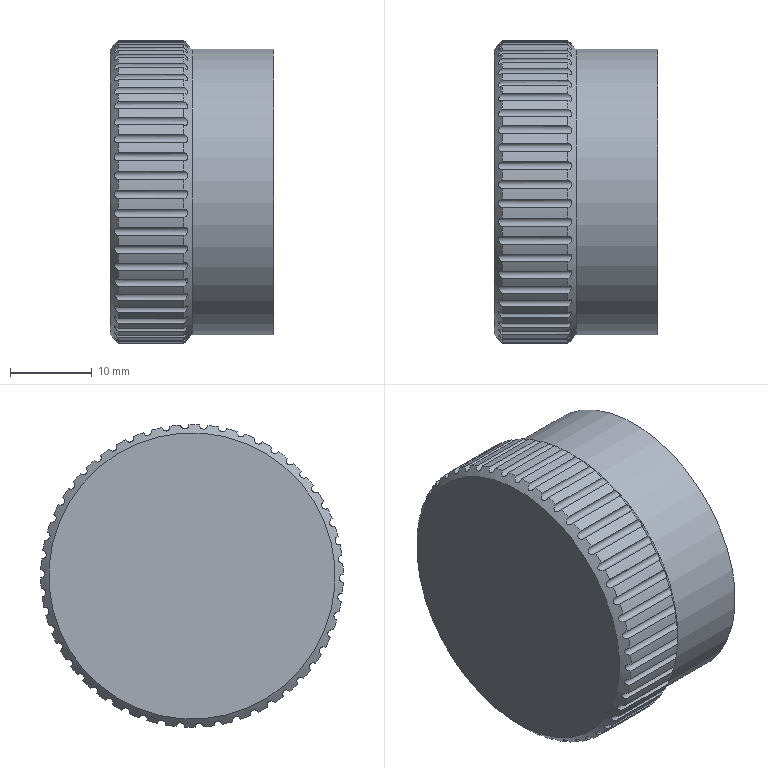Component | NX | 7_OIL_CUP_BODY | 1 solid | 109 faces | volume 7079 mm3 | cylinder 103 | plane 4 | cone 2 | commonest cylinder face diameters 37 x50 1 x50 32 x1 30 x1 35 x1